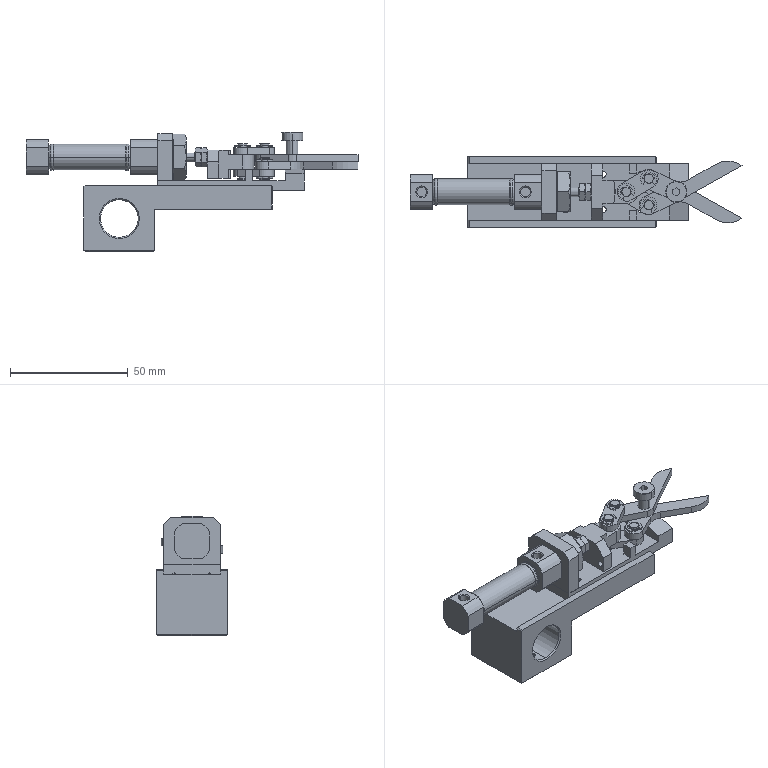Assembly | SolidWorks | mm | 22 component files | 22 solids | 590 faces | box 140.88 x 30 x 50.5 mm | volume 50593 mm3 | cylinder 255 | plane 225 | cone 102 | torus 4 | spline 4 | commonest cylinder face diameters 4 x92 3 x27 2.5 x20 7 x15 8 x12 12 x10 3.4 x10 5.2 x10
Bill of materials:
4ExternalCaliper | 5 |  | Thin flat open ring shaped like an E-style retaining clip: a C-shaped annulus with one wide opening and three inward-pointing prongs whose inner tips have arc-shaped edges
JR-PL-JD-03BasePlate | 1 |  | Rectangular flat plate with nine through holes, two small raised square posts on top, and a stepped/sloped region at one end
JR-PL-JD-04CylinderFixingPlate | 1 |  | Thick rectangular block with two chamfered top corners and one large round through hole in the centre
JR-PL-JD-05ConnectingRod | 2 |  | Flat obround (stadium-shaped) link plate with two round through holes, one at each rounded end
JR-PL-JD-06ConnectingRodPin | 1 |  | Slender solid cylindrical pin with one narrow circumferential groove near each end and small chamfers on both end faces
JR-PL-JD-07Slider | 1 |  | L-profile block: a taller end section with a large transverse through bore and a small cross hole, joined to a long, thinner arm with two parallel through slots and shallow grooves along both top edges
JR-PL-JD-08ConnectingRodPin | 2 |  | Short, thicker solid cylindrical pin with one circumferential groove near each end and chamfered end edges
JR-PL-JD-14FloatingHead | 1 |  | Bracket block with chamfered upper corners, a central channel, two holes in its lower flanges, and a projecting tab with a rounded end and a vertical through hole
JR-PL-JD-15Scissors | 2 |  | Flat bent-shaped plate of constant thickness: a short end with two round through holes, and a longer arm angled away from it that narrows to a curved, pointed tip
SetScrewM4-D5-12 | 1 |  | Shoulder-screw-like fastener: a cylindrical head with a hexagonal socket recess, a long smooth cylindrical shoulder, and a smaller-diameter threaded end with a chamfered tip
Mates:
1. coincident | MI10x10U(0)+()-1/MI 10x10-U_c-1 face at (-19.325, 30.452, 72.77) dir (1, 0, 0) | JR-PL-JD-03BasePlate-1 face at (-19.325, 18.452, 62.77) dir (-1, 0, 0)
2. width | JR-PL-JD-03BasePlate-1 face at (-19.325, 18.452, 62.77) dir (0, -1, 0) | JR-PL-JD-03BasePlate-1 face at (-19.325, 42.452, 62.77) dir (0, 1, 0) | MI10x10U(0)+()-1/MI 10x10-U_c-1 face at (-75.325, 30.452, 72.77) dir (1, 0, 0) r 5.5
3. coincident | JR-PL-JD-03BasePlate-1 face at (-19.325, 18.452, 62.77) dir (0, 0, 1) | JR-PL-JD-04CylinderFixingPlate-1 face at (-19.325, 42.452, 62.77) dir (0, 0, -1)
4. coincident | JR-PL-JD-03BasePlate-1 face at (-19.325, 18.452, 62.77) dir (-1, 0, 0) | JR-PL-JD-04CylinderFixingPlate-1 face at (-19.325, 42.452, 62.77) dir (-1, 0, 0)
5. coincident | JR-PL-JD-03BasePlate-1 face at (-19.325, 18.452, 62.77) dir (0, -1, 0) | JR-PL-JD-04CylinderFixingPlate-1 face at (-19.325, 18.452, 62.77) dir (0, -1, 0)
6. concentric | MI10x10U(0)+()-1/MI 10x10-U_c-1 face at (-19.325, 30.452, 72.77) dir (1, 0, 0) r 6 | JR-PL-JD-04CylinderFixingPlate-1 face at (-13.325, 30.452, 72.77) dir (-1, 0, 0) r 6
7. parallel | MI10x10U(0)+()-1 plane at (-19.325, 30.452, 72.77) dir (0, 0, 1) | JR-PL-JD-03BasePlate-1 face at (-19.325, 18.452, 58.77) dir (0, 0, -1)
8. concentric | MI10x10U(0)+()-1/MI 10x10-U_r-1 face at (-60.294, 30.452, 72.77) dir (1, 0, 0) r 2 | JR-PL-JD-14FloatingHead-1 face at (1.506, 30.452, 72.77) dir (-1, 0, 0) r 1.65
9. distance | MI10x10U(0)+()-1/MI 10x10-U_r-1 face at (-1.494, 30.452, 74.77) dir (-1, 0, 0) | JR-PL-JD-14FloatingHead-1 face at (1.506, 42.452, 75.77) dir (-1, 0, 0)
10. concentric | JR-PL-JD-05ConnectingRod-1 face at (16.506, 30.452, 67.77) dir (0, 0, -1) r 2 | JR-PL-JD-14FloatingHead-1 face at (16.506, 30.452, 75.77) dir (0, 0, 1) r 2
11. concentric | JR-PL-JD-14FloatingHead-1 face at (16.506, 30.452, 75.77) dir (0, 0, 1) r 2 | JR-PL-JD-05ConnectingRod-2 face at (16.506, 30.452, 76.77) dir (0, 0, -1) r 4
12. parallel | JR-PL-JD-03BasePlate-1 face at (-19.325, 18.452, 62.77) dir (0, 0, 1) | JR-PL-JD-14FloatingHead-1 face at (16.506, 30.452, 75.77) dir (0, 0, 1)
13. concentric | JR-PL-JD-03BasePlate-1 face at (37.675, 30.452, 58.77) dir (0, 0, 1) r 1.65 | JR-PL-JD-15Scissors-1 face at (37.675, 30.452, 73.77) dir (0, 0, -1) r 2.55
14. concentric | JR-PL-JD-03BasePlate-1 face at (37.675, 30.452, 58.77) dir (0, 0, 1) r 1.65 | JR-PL-JD-15Scissors-2 face at (37.675, 30.452, 67.77) dir (0, 0, 1) r 2.55
15. concentric | JR-PL-JD-05ConnectingRod-1 face at (25.957, 24.823, 67.77) dir (0, 0, -1) r 2 | JR-PL-JD-15Scissors-2 face at (25.957, 24.823, 67.77) dir (0, 0, 1) r 2.05
16. concentric | JR-PL-JD-05ConnectingRod-2 face at (25.957, 36.081, 76.77) dir (0, 0, -1) r 2 | JR-PL-JD-15Scissors-1 face at (25.957, 36.081, 73.77) dir (0, 0, -1) r 2.05
17. coincident | JR-PL-JD-05ConnectingRod-1 face at (16.506, 30.452, 67.77) dir (0, 0, 1) | JR-PL-JD-15Scissors-2 face at (39.513, 20.242, 67.77) dir (0, 0, -1)
18. coincident | JR-PL-JD-05ConnectingRod-2 face at (16.506, 30.452, 73.77) dir (0, 0, -1) | JR-PL-JD-15Scissors-1 face at (39.513, 40.663, 73.77) dir (0, 0, 1)
19. coincident | JR-PL-JD-15Scissors-1 face at (39.513, 40.663, 70.77) dir (0, 0, -1) | JR-PL-JD-15Scissors-2 face at (39.513, 20.242, 70.77) dir (0, 0, 1)
20. coincident | 4ExternalCaliper-1 face at (25.957, 36.081, 77.72) dir (0, 0, 1) | JR-PL-JD-08ConnectingRodPin-2 face at (25.957, 38.081, 77.72) dir (0, 0, -1)
21. concentric | JR-PL-JD-05ConnectingRod-2 face at (25.957, 36.081, 76.77) dir (0, 0, -1) r 2 | 4ExternalCaliper-1 face at (25.957, 36.081, 77.72) dir (0, 0, 1) r 1.5
22. coincident | 4ExternalCaliper-2 face at (25.957, 36.081, 69.82) dir (0, 0, -1) | JR-PL-JD-08ConnectingRodPin-2 face at (25.957, 38.081, 69.82) dir (0, 0, 1)
23. concentric | JR-PL-JD-15Scissors-1 face at (25.957, 36.081, 73.77) dir (0, 0, -1) r 2.05 | 4ExternalCaliper-2 face at (25.957, 36.081, 70.42) dir (0, 0, 1) r 1.5
24. concentric | JR-PL-JD-15Scissors-2 face at (25.957, 24.823, 67.77) dir (0, 0, 1) r 2.05 | 4ExternalCaliper-3 face at (25.957, 24.823, 71.62) dir (0, 0, 1) r 1.5
25. concentric | JR-PL-JD-05ConnectingRod-1 face at (25.957, 24.823, 67.77) dir (0, 0, -1) r 2 | 4ExternalCaliper-4 face at (25.957, 24.823, 64.52) dir (0, 0, 1) r 1.5
26. concentric | 4ExternalCaliper-5 face at (16.506, 30.452, 77.12) dir (0, 0, -1) r 1.5 | JR-PL-JD-05ConnectingRod-2 face at (16.506, 30.452, 76.77) dir (0, 0, -1) r 2
27. coincident | 4ExternalCaliper-5 face at (16.506, 30.452, 77.72) dir (0, 0, 1) | JR-PL-JD-06ConnectingRodPin-1 face at (16.506, 32.452, 77.72) dir (0, 0, -1)
28. concentric | JR-PL-JD-15Scissors-2 face at (25.957, 24.823, 67.77) dir (0, 0, 1) r 2.05 | JR-PL-JD-08ConnectingRodPin-1 face at (25.957, 24.823, 63.02) dir (0, 0, -1) r 2
29. width | JR-PL-JD-15Scissors-2 face at (39.513, 20.242, 70.77) dir (0, 0, 1) | JR-PL-JD-05ConnectingRod-1 face at (16.506, 30.452, 64.77) dir (0, 0, -1) | JR-PL-JD-08ConnectingRodPin-1 face at (25.957, 24.823, 72.52) dir (0, 0, 1) | JR-PL-JD-08ConnectingRodPin-1 face at (25.957, 24.823, 63.02) dir (0, 0, -1)
30. concentric | JR-PL-JD-05ConnectingRod-2 face at (25.957, 36.081, 76.77) dir (0, 0, -1) r 2 | JR-PL-JD-08ConnectingRodPin-2 face at (25.957, 36.081, 69.02) dir (0, 0, -1) r 2
31. width | JR-PL-JD-05ConnectingRod-2 face at (16.506, 30.452, 76.77) dir (0, 0, 1) | JR-PL-JD-15Scissors-1 face at (39.513, 40.663, 70.77) dir (0, 0, -1) | JR-PL-JD-08ConnectingRodPin-2 face at (25.957, 36.081, 78.52) dir (0, 0, 1) | JR-PL-JD-08ConnectingRodPin-2 face at (25.957, 36.081, 69.02) dir (0, 0, -1)
32. concentric | JR-PL-JD-14FloatingHead-1 face at (16.506, 30.452, 75.77) dir (0, 0, 1) r 2 | JR-PL-JD-06ConnectingRodPin-1 face at (16.506, 30.452, 63.02) dir (0, 0, -1) r 2
33. width | JR-PL-JD-06ConnectingRodPin-1 face at (16.506, 30.452, 78.52) dir (0, 0, 1) | JR-PL-JD-06ConnectingRodPin-1 face at (16.506, 30.452, 63.02) dir (0, 0, -1) | JR-PL-JD-05ConnectingRod-2 face at (16.506, 30.452, 76.77) dir (0, 0, 1) | JR-PL-JD-05ConnectingRod-1 face at (16.506, 30.452, 64.77) dir (0, 0, -1)
34. distance | JR-PL-JD-15Scissors-2 face at (39.513, 20.242, 67.77) dir (0, 0, -1) | JR-PL-JD-03BasePlate-1 face at (-19.325, 18.452, 62.77) dir (0, 0, 1)
35. coincident | JR-PL-JD-03BasePlate-1 face at (-19.325, 18.452, 58.77) dir (0, 0, -1) | JR-PL-JD-07Slider-1 face at (-50.739, 18.452, 58.77) dir (0, 0, 1)
36. coincident | JR-PL-JD-03BasePlate-1 face at (-19.325, 42.452, 62.77) dir (0, 1, 0) | JR-PL-JD-07Slider-1 face at (-50.739, 42.452, 60.77) dir (0, -1, 0)
37. coincident | JR-PL-JD-03BasePlate-1 face at (-19.325, 18.452, 67.77) dir (0, 0, 1) | SetScrewM4-D5-12-1 face at (39.675, 30.452, 67.77) dir (0, 0, -1)
38. concentric | JR-PL-JD-15Scissors-1 face at (37.675, 30.452, 73.77) dir (0, 0, -1) r 2.55 | SetScrewM4-D5-12-1 face at (37.675, 30.452, 59.77) dir (0, 0, -1) r 2.5
39. coincident | 4ExternalCaliper-3 face at (25.957, 24.823, 71.02) dir (0, 0, -1) | JR-PL-JD-08ConnectingRodPin-1 face at (25.957, 26.323, 71.02) dir (0, 0, 1)
40. coincident | 4ExternalCaliper-4 face at (25.957, 24.823, 64.52) dir (0, 0, 1) | JR-PL-JD-08ConnectingRodPin-1 face at (25.957, 26.323, 64.52) dir (0, 0, -1)
41. coincident | MI 10x10-U_c-1 axis at (-80.9, 0, 0) dir (1, 0, 0) | MI 10x10-U_r-1 axis at (80.9, 0, 0) dir (-1, 0, 0)
42. angle | MI 10x10-U_r-1 plane at (0, 0, 0) dir (0, 0, -1) | MI 10x10-U_c-1 plane at (0, 0, 0) dir (0, 0, -1)
43. coincident | MI 10x10-U_r-1 axis at (-80.9, 0, 0) dir (1, 0, 0) | MI10-M4x0_7 - Nut-1 axis at (65.391, 0, 0) dir (-1, 0, 0)
44. angle | MI10-M4x0_7 - Nut-1 plane at (-15.509, 0, 0) dir (0, 0, -1) | MI 10x10-U_r-1 plane at (0, 0, 0) dir (0, 0, -1)
45. coincident | MI 10x10-U_r-1 axis at (-80.9, 0, 0) dir (1, 0, 0) | MI10-M4x0_7 - Nut-2 axis at (62.891, 0, 0) dir (-1, 0, 0)
46. angle | MI10-M4x0_7 - Nut-2 plane at (-18.009, 0, 0) dir (0, 0, -1) | MI 10x10-U_r-1 plane at (0, 0, 0) dir (0, 0, -1)
47. distance | MI10-M12x1_25 - Nut-1 plane at (-6, 0, 0) dir (1, 0, 0) | MI 10x10-U_c-1 plane at (0, 0, 0) dir (-1, 0, 0)
48. coincident | MI 10x10-U_c-1 axis at (-80.9, 0, 0) dir (1, 0, 0) | MI10-M12x1_25 - Nut-1 axis at (68.9, 0, 0) dir (-1, 0, 0)
49. angle | MI10-M12x1_25 - Nut-1 plane at (-12, 0, 0) dir (0, 0, -1) | MI 10x10-U_c-1 plane at (0, 0, 0) dir (0, 0, -1)
50. distance | MI 10x10-U_c-1 face at (-12, 0, 0) dir (-1, 0, 0) | MI 10x10-U_r-1 face at (-28, 0, 0) dir (-1, 0, 0)